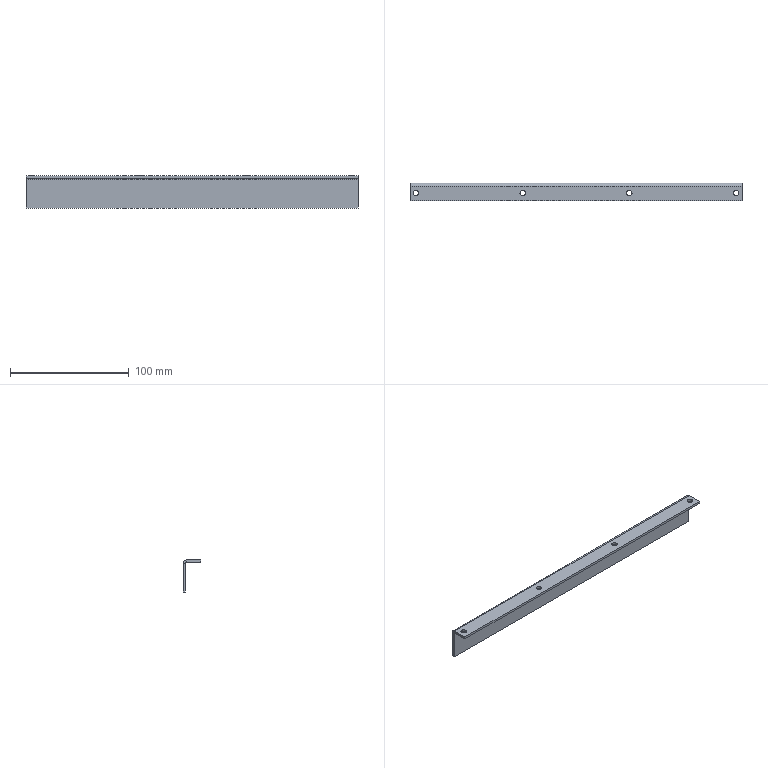Component | SolidWorks | P-SLJ-001-002-1 | 1 solid | 22 faces | box 280 x 15 x 27 mm | volume 21855 mm3 | plane 12 | cylinder 10 | commonest cylinder face diameters 4.5 x8 5.473 x1 1.473 x1 | material SUS 304
STEP:
#1=COLOUR_RGB('',0.7922,0.8196,0.9333);
#2=FILL_AREA_STYLE_COLOUR('',#1);
#3=FILL_AREA_STYLE('',(#2));
#4=SURFACE_STYLE_FILL_AREA(#3);
#5=SURFACE_SIDE_STYLE('',(#4));
#6=SURFACE_STYLE_USAGE(.BOTH.,#5);
#7=PRESENTATION_STYLE_ASSIGNMENT((#6));
#8=CARTESIAN_POINT('',(8.415,-2.579,48.253));
#9=VERTEX_POINT('',#8);
#10=CARTESIAN_POINT('',(8.238,-2.579,48.253));
#11=VERTEX_POINT('',#10);
#12=CARTESIAN_POINT('',(8.327,-2.579,48.253));
#13=DIRECTION('',(0.,0.,-1.));
#14=DIRECTION('',(-1.,0.,0.));
#15=AXIS2_PLACEMENT_3D('',#12,#13,#14);
#16=CIRCLE('',#15,0.08858);
#17=EDGE_CURVE('',#9,#11,#16,.T.);
#18=ORIENTED_EDGE('',*,*,#17,.F.);
#19=CARTESIAN_POINT('',(8.415,-2.579,48.175));
#20=VERTEX_POINT('',#19);
#21=CARTESIAN_POINT('',(8.415,-2.579,48.175));
#22=DIRECTION('',(0.,0.,-1.));
#23=VECTOR('',#22,39.37);
#24=LINE('',#21,#23);
#25=EDGE_CURVE('',#9,#20,#24,.T.);
#26=ORIENTED_EDGE('',*,*,#25,.T.);
#27=CARTESIAN_POINT('',(8.238,-2.579,48.175));
#28=VERTEX_POINT('',#27);
#29=CARTESIAN_POINT('',(8.327,-2.579,48.175));
#30=DIRECTION('',(0.,0.,-1.));
#31=DIRECTION('',(-1.,0.,0.));
#32=AXIS2_PLACEMENT_3D('',#29,#30,#31);
#33=CIRCLE('',#32,0.08858);
#34=EDGE_CURVE('',#20,#28,#33,.T.);
#35=ORIENTED_EDGE('',*,*,#34,.T.);
#36=CARTESIAN_POINT('',(8.238,-2.579,48.175));
#37=DIRECTION('',(0.,0.,-1.));
#38=VECTOR('',#37,39.37);
#39=LINE('',#36,#38);
#40=EDGE_CURVE('',#11,#28,#39,.T.);
#41=ORIENTED_EDGE('',*,*,#40,.F.);
#42=EDGE_LOOP('',(#18,#26,#35,#41));
#43=FACE_OUTER_BOUND('',#42,.T.);
#44=CARTESIAN_POINT('',(8.327,-2.579,48.175));
#45=DIRECTION('',(0.,0.,-1.));
#46=DIRECTION('',(-1.,0.,0.));
#47=AXIS2_PLACEMENT_3D('',#44,#45,#46);
#48=CYLINDRICAL_SURFACE('',#47,0.08858);
#49=ADVANCED_FACE('',(#43),#48,.F.);
#50=CARTESIAN_POINT('',(4.872,-2.579,48.253));
#51=VERTEX_POINT('',#50);
#52=CARTESIAN_POINT('',(4.695,-2.579,48.253));
#53=VERTEX_POINT('',#52);
#54=CARTESIAN_POINT('',(4.783,-2.579,48.253));
#55=DIRECTION('',(0.,0.,-1.));
#56=DIRECTION('',(-1.,0.,0.));
#57=AXIS2_PLACEMENT_3D('',#54,#55,#56);
#58=CIRCLE('',#57,0.08858);
#59=EDGE_CURVE('',#51,#53,#58,.T.);
#60=ORIENTED_EDGE('',*,*,#59,.F.);
#61=CARTESIAN_POINT('',(4.872,-2.579,48.175));
#62=VERTEX_POINT('',#61);
#63=CARTESIAN_POINT('',(4.872,-2.579,48.175));
#64=DIRECTION('',(0.,0.,-1.));
#65=VECTOR('',#64,39.37);
#66=LINE('',#63,#65);
#67=EDGE_CURVE('',#51,#62,#66,.T.);
#68=ORIENTED_EDGE('',*,*,#67,.T.);
#69=CARTESIAN_POINT('',(4.695,-2.579,48.175));
#70=VERTEX_POINT('',#69);
#71=CARTESIAN_POINT('',(4.783,-2.579,48.175));
#72=DIRECTION('',(0.,0.,-1.));
#73=DIRECTION('',(-1.,0.,0.));
#74=AXIS2_PLACEMENT_3D('',#71,#72,#73);
#75=CIRCLE('',#74,0.08858);
#76=EDGE_CURVE('',#62,#70,#75,.T.);
#77=ORIENTED_EDGE('',*,*,#76,.T.);
#78=CARTESIAN_POINT('',(4.695,-2.579,48.175));
#79=DIRECTION('',(0.,0.,-1.));
#80=VECTOR('',#79,39.37);
#81=LINE('',#78,#80);
#82=EDGE_CURVE('',#53,#70,#81,.T.);
#83=ORIENTED_EDGE('',*,*,#82,.F.);
#84=EDGE_LOOP('',(#60,#68,#77,#83));
#85=FACE_OUTER_BOUND('',#84,.T.);
#86=CARTESIAN_POINT('',(4.783,-2.579,48.175));
#87=DIRECTION('',(0.,0.,-1.));
#88=DIRECTION('',(-1.,0.,0.));
#89=AXIS2_PLACEMENT_3D('',#86,#87,#88);
#90=CYLINDRICAL_SURFACE('',#89,0.08858);
#91=ADVANCED_FACE('',(#85),#90,.F.);
#92=CARTESIAN_POINT('',(1.329,-2.579,48.253));
#93=VERTEX_POINT('',#92);
#94=CARTESIAN_POINT('',(1.152,-2.579,48.253));
#95=VERTEX_POINT('',#94);
#96=CARTESIAN_POINT('',(1.24,-2.579,48.253));
#97=DIRECTION('',(0.,0.,-1.));
#98=DIRECTION('',(-1.,0.,0.));
#99=AXIS2_PLACEMENT_3D('',#96,#97,#98);
#100=CIRCLE('',#99,0.08858);
#101=EDGE_CURVE('',#93,#95,#100,.T.);
#102=ORIENTED_EDGE('',*,*,#101,.F.);
#103=CARTESIAN_POINT('',(1.329,-2.579,48.175));
#104=VERTEX_POINT('',#103);
#105=CARTESIAN_POINT('',(1.329,-2.579,48.175));
#106=DIRECTION('',(0.,0.,-1.));
#107=VECTOR('',#106,39.37);
#108=LINE('',#105,#107);
#109=EDGE_CURVE('',#93,#104,#108,.T.);
#110=ORIENTED_EDGE('',*,*,#109,.T.);
#111=CARTESIAN_POINT('',(1.152,-2.579,48.175));
#112=VERTEX_POINT('',#111);
#113=CARTESIAN_POINT('',(1.24,-2.579,48.175));
#114=DIRECTION('',(0.,0.,-1.));
#115=DIRECTION('',(-1.,0.,0.));
#116=AXIS2_PLACEMENT_3D('',#113,#114,#115);
#117=CIRCLE('',#116,0.08858);
#118=EDGE_CURVE('',#104,#112,#117,.T.);
#119=ORIENTED_EDGE('',*,*,#118,.T.);
#120=CARTESIAN_POINT('',(1.152,-2.579,48.175));
#121=DIRECTION('',(0.,0.,-1.));
#122=VECTOR('',#121,39.37);
#123=LINE('',#120,#122);
#124=EDGE_CURVE('',#95,#112,#123,.T.);
#125=ORIENTED_EDGE('',*,*,#124,.F.);
#126=EDGE_LOOP('',(#102,#110,#119,#125));
#127=FACE_OUTER_BOUND('',#126,.T.);
#128=CARTESIAN_POINT('',(1.24,-2.579,48.175));
#129=DIRECTION('',(0.,0.,-1.));
#130=DIRECTION('',(-1.,0.,0.));
#131=AXIS2_PLACEMENT_3D('',#128,#129,#130);
#132=CYLINDRICAL_SURFACE('',#131,0.08858);
#133=ADVANCED_FACE('',(#127),#132,.F.);
#134=CARTESIAN_POINT('',(-2.215,-2.579,48.253));
#135=VERTEX_POINT('',#134);
#136=CARTESIAN_POINT('',(-2.392,-2.579,48.253));
#137=VERTEX_POINT('',#136);
#138=CARTESIAN_POINT('',(-2.303,-2.579,48.253));
#139=DIRECTION('',(0.,0.,-1.));
#140=DIRECTION('',(-1.,0.,0.));
#141=AXIS2_PLACEMENT_3D('',#138,#139,#140);
#142=CIRCLE('',#141,0.08858);
#143=EDGE_CURVE('',#135,#137,#142,.T.);
#144=ORIENTED_EDGE('',*,*,#143,.F.);
#145=CARTESIAN_POINT('',(-2.215,-2.579,48.175));
#146=VERTEX_POINT('',#145);
#147=CARTESIAN_POINT('',(-2.215,-2.579,48.175));
#148=DIRECTION('',(0.,0.,-1.));
#149=VECTOR('',#148,39.37);
#150=LINE('',#147,#149);
#151=EDGE_CURVE('',#135,#146,#150,.T.);
#152=ORIENTED_EDGE('',*,*,#151,.T.);
#153=CARTESIAN_POINT('',(-2.392,-2.579,48.175));
#154=VERTEX_POINT('',#153);
#155=CARTESIAN_POINT('',(-2.303,-2.579,48.175));
#156=DIRECTION('',(0.,0.,-1.));
#157=DIRECTION('',(-1.,0.,0.));
#158=AXIS2_PLACEMENT_3D('',#155,#156,#157);
#159=CIRCLE('',#158,0.08858);
#160=EDGE_CURVE('',#146,#154,#159,.T.);
#161=ORIENTED_EDGE('',*,*,#160,.T.);
#162=CARTESIAN_POINT('',(-2.392,-2.579,48.175));
#163=DIRECTION('',(0.,0.,-1.));
#164=VECTOR('',#163,39.37);
#165=LINE('',#162,#164);
#166=EDGE_CURVE('',#137,#154,#165,.T.);
#167=ORIENTED_EDGE('',*,*,#166,.F.);
#168=EDGE_LOOP('',(#144,#152,#161,#167));
#169=FACE_OUTER_BOUND('',#168,.T.);
#170=CARTESIAN_POINT('',(-2.303,-2.579,48.175));
#171=DIRECTION('',(0.,0.,-1.));
#172=DIRECTION('',(-1.,0.,0.));
#173=AXIS2_PLACEMENT_3D('',#170,#171,#172);
#174=CYLINDRICAL_SURFACE('',#173,0.08858);
#175=ADVANCED_FACE('',(#169),#174,.F.);
#176=CARTESIAN_POINT('',(8.524,-2.352,48.175));
#177=VERTEX_POINT('',#176);
#178=CARTESIAN_POINT('',(8.524,-2.835,48.175));
#179=VERTEX_POINT('',#178);
#180=CARTESIAN_POINT('',(8.524,-2.835,48.175));
#181=DIRECTION('',(-0.,-1.,0.));
#182=VECTOR('',#181,39.37);
#183=LINE('',#180,#182);
#184=EDGE_CURVE('',#177,#179,#183,.T.);
#185=ORIENTED_EDGE('',*,*,#184,.F.);
#186=CARTESIAN_POINT('',(8.524,-2.352,48.253));
#187=VERTEX_POINT('',#186);
#188=CARTESIAN_POINT('',(8.524,-2.352,48.175));
#189=DIRECTION('',(0.,0.,1.));
#190=VECTOR('',#189,39.37);
#191=LINE('',#188,#190);
#192=EDGE_CURVE('',#177,#187,#191,.T.);
#193=ORIENTED_EDGE('',*,*,#192,.T.);
#194=CARTESIAN_POINT('',(8.524,-2.835,48.253));
#195=VERTEX_POINT('',#194);
#196=CARTESIAN_POINT('',(8.524,-2.835,48.253));
#197=DIRECTION('',(-0.,-1.,0.));
#198=VECTOR('',#197,39.37);
#199=LINE('',#196,#198);
#200=EDGE_CURVE('',#187,#195,#199,.T.);
#201=ORIENTED_EDGE('',*,*,#200,.T.);
#202=CARTESIAN_POINT('',(8.524,-2.835,48.253));
#203=DIRECTION('',(0.,0.,-1.));
#204=VECTOR('',#203,39.37);
#205=LINE('',#202,#204);
#206=EDGE_CURVE('',#195,#179,#205,.T.);
#207=ORIENTED_EDGE('',*,*,#206,.T.);
#208=EDGE_LOOP('',(#185,#193,#201,#207));
#209=FACE_OUTER_BOUND('',#208,.T.);
#210=CARTESIAN_POINT('',(8.524,-2.835,48.253));
#211=DIRECTION('',(1.,-0.,0.));
#212=DIRECTION('',(0.,0.,-1.));
#213=AXIS2_PLACEMENT_3D('',#210,#211,#212);
#214=PLANE('',#213);
#215=ADVANCED_FACE('',(#209),#214,.T.);
#216=CARTESIAN_POINT('',(8.327,-2.579,48.253));
#217=DIRECTION('',(0.,0.,-1.));
#218=DIRECTION('',(-1.,0.,0.));
#219=AXIS2_PLACEMENT_3D('',#216,#217,#218);
#220=CIRCLE('',#219,0.08858);
#221=EDGE_CURVE('',#11,#9,#220,.T.);
#222=ORIENTED_EDGE('',*,*,#221,.T.);
#223=ORIENTED_EDGE('',*,*,#17,.T.);
#224=EDGE_LOOP('',(#222,#223));
#225=FACE_BOUND('',#224,.T.);
#226=CARTESIAN_POINT('',(4.783,-2.579,48.253));
#227=DIRECTION('',(0.,0.,-1.));
#228=DIRECTION('',(-1.,0.,0.));
#229=AXIS2_PLACEMENT_3D('',#226,#227,#228);
#230=CIRCLE('',#229,0.08858);
#231=EDGE_CURVE('',#53,#51,#230,.T.);
#232=ORIENTED_EDGE('',*,*,#231,.T.);
#233=ORIENTED_EDGE('',*,*,#59,.T.);
#234=EDGE_LOOP('',(#232,#233));
#235=FACE_BOUND('',#234,.T.);
#236=CARTESIAN_POINT('',(1.24,-2.579,48.253));
#237=DIRECTION('',(0.,0.,-1.));
#238=DIRECTION('',(-1.,0.,0.));
#239=AXIS2_PLACEMENT_3D('',#236,#237,#238);
#240=CIRCLE('',#239,0.08858);
#241=EDGE_CURVE('',#95,#93,#240,.T.);
#242=ORIENTED_EDGE('',*,*,#241,.T.);
#243=ORIENTED_EDGE('',*,*,#101,.T.);
#244=EDGE_LOOP('',(#242,#243));
#245=FACE_BOUND('',#244,.T.);
#246=CARTESIAN_POINT('',(-2.303,-2.579,48.253));
#247=DIRECTION('',(0.,0.,-1.));
#248=DIRECTION('',(-1.,0.,0.));
#249=AXIS2_PLACEMENT_3D('',#246,#247,#248);
#250=CIRCLE('',#249,0.08858);
#251=EDGE_CURVE('',#137,#135,#250,.T.);
#252=ORIENTED_EDGE('',*,*,#251,.T.);
#253=ORIENTED_EDGE('',*,*,#143,.T.);
#254=EDGE_LOOP('',(#252,#253));
#255=FACE_BOUND('',#254,.T.);
#256=ORIENTED_EDGE('',*,*,#200,.F.);
#257=CARTESIAN_POINT('',(-2.5,-2.352,48.253));
#258=VERTEX_POINT('',#257);
#259=CARTESIAN_POINT('',(8.524,-2.352,48.253));
#260=DIRECTION('',(-1.,0.,0.));
#261=VECTOR('',#260,39.37);
#262=LINE('',#259,#261);
#263=EDGE_CURVE('',#187,#258,#262,.T.);
#264=ORIENTED_EDGE('',*,*,#263,.T.);
#265=CARTESIAN_POINT('',(-2.5,-2.835,48.253));
#266=VERTEX_POINT('',#265);
#267=CARTESIAN_POINT('',(-2.5,-2.835,48.253));
#268=DIRECTION('',(0.,1.,0.));
#269=VECTOR('',#268,39.37);
#270=LINE('',#267,#269);
#271=EDGE_CURVE('',#266,#258,#270,.T.);
#272=ORIENTED_EDGE('',*,*,#271,.F.);
#273=CARTESIAN_POINT('',(8.524,-2.835,48.253));
#274=DIRECTION('',(-1.,0.,0.));
#275=VECTOR('',#274,39.37);
#276=LINE('',#273,#275);
#277=EDGE_CURVE('',#195,#266,#276,.T.);
#278=ORIENTED_EDGE('',*,*,#277,.F.);
#279=EDGE_LOOP('',(#256,#264,#272,#278));
#280=FACE_OUTER_BOUND('',#279,.T.);
#281=CARTESIAN_POINT('',(3.012,-2.579,48.253));
#282=DIRECTION('',(0.,0.,1.));
#283=DIRECTION('',(1.,-0.,0.));
#284=AXIS2_PLACEMENT_3D('',#281,#282,#283);
#285=PLANE('',#284);
#286=ADVANCED_FACE('',(#225,#235,#245,#255,#280),#285,.T.);
#287=CARTESIAN_POINT('',(8.327,-2.579,48.175));
#288=DIRECTION('',(0.,0.,-1.));
#289=DIRECTION('',(-1.,0.,0.));
#290=AXIS2_PLACEMENT_3D('',#287,#288,#289);
#291=CIRCLE('',#290,0.08858);
#292=EDGE_CURVE('',#28,#20,#291,.T.);
#293=ORIENTED_EDGE('',*,*,#292,.F.);
#294=ORIENTED_EDGE('',*,*,#34,.F.);
#295=EDGE_LOOP('',(#293,#294));
#296=FACE_BOUND('',#295,.T.);
#297=CARTESIAN_POINT('',(4.783,-2.579,48.175));
#298=DIRECTION('',(0.,0.,-1.));
#299=DIRECTION('',(-1.,0.,0.));
#300=AXIS2_PLACEMENT_3D('',#297,#298,#299);
#301=CIRCLE('',#300,0.08858);
#302=EDGE_CURVE('',#70,#62,#301,.T.);
#303=ORIENTED_EDGE('',*,*,#302,.F.);
#304=ORIENTED_EDGE('',*,*,#76,.F.);
#305=EDGE_LOOP('',(#303,#304));
#306=FACE_BOUND('',#305,.T.);
#307=CARTESIAN_POINT('',(1.24,-2.579,48.175));
#308=DIRECTION('',(0.,0.,-1.));
#309=DIRECTION('',(-1.,0.,0.));
#310=AXIS2_PLACEMENT_3D('',#307,#308,#309);
#311=CIRCLE('',#310,0.08858);
#312=EDGE_CURVE('',#112,#104,#311,.T.);
#313=ORIENTED_EDGE('',*,*,#312,.F.);
#314=ORIENTED_EDGE('',*,*,#118,.F.);
#315=EDGE_LOOP('',(#313,#314));
#316=FACE_BOUND('',#315,.T.);
#317=CARTESIAN_POINT('',(-2.303,-2.579,48.175));
#318=DIRECTION('',(0.,0.,-1.));
#319=DIRECTION('',(-1.,0.,0.));
#320=AXIS2_PLACEMENT_3D('',#317,#318,#319);
#321=CIRCLE('',#320,0.08858);
#322=EDGE_CURVE('',#154,#146,#321,.T.);
#323=ORIENTED_EDGE('',*,*,#322,.F.);
#324=ORIENTED_EDGE('',*,*,#160,.F.);
#325=EDGE_LOOP('',(#323,#324));
#326=FACE_BOUND('',#325,.T.);
#327=CARTESIAN_POINT('',(-2.5,-2.352,48.175));
#328=VERTEX_POINT('',#327);
#329=CARTESIAN_POINT('',(8.524,-2.352,48.175));
#330=DIRECTION('',(-1.,0.,0.));
#331=VECTOR('',#330,39.37);
#332=LINE('',#329,#331);
#333=EDGE_CURVE('',#177,#328,#332,.T.);
#334=ORIENTED_EDGE('',*,*,#333,.F.);
#335=ORIENTED_EDGE('',*,*,#184,.T.);
#336=CARTESIAN_POINT('',(-2.5,-2.835,48.175));
#337=VERTEX_POINT('',#336);
#338=CARTESIAN_POINT('',(8.524,-2.835,48.175));
#339=DIRECTION('',(-1.,0.,0.));
#340=VECTOR('',#339,39.37);
#341=LINE('',#338,#340);
#342=EDGE_CURVE('',#179,#337,#341,.T.);
#343=ORIENTED_EDGE('',*,*,#342,.T.);
#344=CARTESIAN_POINT('',(-2.5,-2.835,48.175));
#345=DIRECTION('',(0.,1.,0.));
#346=VECTOR('',#345,39.37);
#347=LINE('',#344,#346);
#348=EDGE_CURVE('',#337,#328,#347,.T.);
#349=ORIENTED_EDGE('',*,*,#348,.T.);
#350=EDGE_LOOP('',(#334,#335,#343,#349));
#351=FACE_OUTER_BOUND('',#350,.T.);
#352=CARTESIAN_POINT('',(3.012,-2.579,48.175));
#353=DIRECTION('',(0.,0.,1.));
#354=DIRECTION('',(1.,-0.,0.));
#355=AXIS2_PLACEMENT_3D('',#352,#353,#354);
#356=PLANE('',#355);
#357=ADVANCED_FACE('',(#296,#306,#316,#326,#351),#356,.F.);
#358=CARTESIAN_POINT('',(-2.5,-2.352,48.175));
#359=DIRECTION('',(0.,0.,1.));
#360=VECTOR('',#359,39.37);
#361=LINE('',#358,#360);
#362=EDGE_CURVE('',#328,#258,#361,.T.);
#363=ORIENTED_EDGE('',*,*,#362,.F.);
#364=ORIENTED_EDGE('',*,*,#348,.F.);
#365=CARTESIAN_POINT('',(-2.5,-2.835,48.253));
#366=DIRECTION('',(0.,0.,-1.));
#367=VECTOR('',#366,39.37);
#368=LINE('',#365,#367);
#369=EDGE_CURVE('',#266,#337,#368,.T.);
#370=ORIENTED_EDGE('',*,*,#369,.F.);
#371=ORIENTED_EDGE('',*,*,#271,.T.);
#372=EDGE_LOOP('',(#363,#364,#370,#371));
#373=FACE_OUTER_BOUND('',#372,.T.);
#374=CARTESIAN_POINT('',(-2.5,-2.835,48.253));
#375=DIRECTION('',(-1.,0.,0.));
#376=DIRECTION('',(0.,0.,1.));
#377=AXIS2_PLACEMENT_3D('',#374,#375,#376);
#378=PLANE('',#377);
#379=ADVANCED_FACE('',(#373),#378,.T.);
#380=ORIENTED_EDGE('',*,*,#342,.F.);
#381=ORIENTED_EDGE('',*,*,#206,.F.);
#382=ORIENTED_EDGE('',*,*,#277,.T.);
#383=ORIENTED_EDGE('',*,*,#369,.T.);
#384=EDGE_LOOP('',(#380,#381,#382,#383));
#385=FACE_OUTER_BOUND('',#384,.T.);
#386=CARTESIAN_POINT('',(8.524,-2.835,48.253));
#387=DIRECTION('',(-0.,-1.,0.));
#388=DIRECTION('',(-1.,0.,0.));
#389=AXIS2_PLACEMENT_3D('',#386,#387,#388);
#390=PLANE('',#389);
#391=ADVANCED_FACE('',(#385),#390,.T.);
#392=CARTESIAN_POINT('',(-2.5,-2.323,48.146));
#393=VERTEX_POINT('',#392);
#394=CARTESIAN_POINT('',(-2.5,-2.244,48.146));
#395=VERTEX_POINT('',#394);
#396=CARTESIAN_POINT('',(-2.5,-2.323,48.146));
#397=DIRECTION('',(0.,1.,0.));
#398=VECTOR('',#397,39.37);
#399=LINE('',#396,#398);
#400=EDGE_CURVE('',#393,#395,#399,.T.);
#401=ORIENTED_EDGE('',*,*,#400,.F.);
#402=CARTESIAN_POINT('',(-2.5,-2.352,48.146));
#403=DIRECTION('',(-1.,0.,0.));
#404=DIRECTION('',(0.,0.,-1.));
#405=AXIS2_PLACEMENT_3D('',#402,#403,#404);
#406=CIRCLE('',#405,0.029);
#407=EDGE_CURVE('',#328,#393,#406,.T.);
#408=ORIENTED_EDGE('',*,*,#407,.F.);
#409=ORIENTED_EDGE('',*,*,#362,.T.);
#410=CARTESIAN_POINT('',(-2.5,-2.352,48.146));
#411=DIRECTION('',(-1.,0.,0.));
#412=DIRECTION('',(0.,0.,-1.));
#413=AXIS2_PLACEMENT_3D('',#410,#411,#412);
#414=CIRCLE('',#413,0.1077);
#415=EDGE_CURVE('',#258,#395,#414,.T.);
#416=ORIENTED_EDGE('',*,*,#415,.T.);
#417=EDGE_LOOP('',(#401,#408,#409,#416));
#418=FACE_OUTER_BOUND('',#417,.T.);
#419=CARTESIAN_POINT('',(-2.5,-2.352,48.146));
#420=DIRECTION('',(-1.,0.,0.));
#421=DIRECTION('',(0.,0.,1.));
#422=AXIS2_PLACEMENT_3D('',#419,#420,#421);
#423=PLANE('',#422);
#424=ADVANCED_FACE('',(#418),#423,.T.);
#425=CARTESIAN_POINT('',(8.524,-2.323,48.146));
#426=VERTEX_POINT('',#425);
#427=CARTESIAN_POINT('',(8.524,-2.352,48.146));
#428=DIRECTION('',(1.,-0.,0.));
#429=DIRECTION('',(0.,0.,-1.));
#430=AXIS2_PLACEMENT_3D('',#427,#428,#429);
#431=CIRCLE('',#430,0.029);
#432=EDGE_CURVE('',#426,#177,#431,.T.);
#433=ORIENTED_EDGE('',*,*,#432,.F.);
#434=CARTESIAN_POINT('',(8.524,-2.244,48.146));
#435=VERTEX_POINT('',#434);
#436=CARTESIAN_POINT('',(8.524,-2.323,48.146));
#437=DIRECTION('',(0.,1.,0.));
#438=VECTOR('',#437,39.37);
#439=LINE('',#436,#438);
#440=EDGE_CURVE('',#426,#435,#439,.T.);
#441=ORIENTED_EDGE('',*,*,#440,.T.);
#442=CARTESIAN_POINT('',(8.524,-2.352,48.146));
#443=DIRECTION('',(1.,-0.,0.));
#444=DIRECTION('',(0.,0.,-1.));
#445=AXIS2_PLACEMENT_3D('',#442,#443,#444);
#446=CIRCLE('',#445,0.1077);
#447=EDGE_CURVE('',#435,#187,#446,.T.);
#448=ORIENTED_EDGE('',*,*,#447,.T.);
#449=ORIENTED_EDGE('',*,*,#192,.F.);
#450=EDGE_LOOP('',(#433,#441,#448,#449));
#451=FACE_OUTER_BOUND('',#450,.T.);
#452=CARTESIAN_POINT('',(8.524,-2.352,48.146));
#453=DIRECTION('',(-1.,0.,0.));
#454=DIRECTION('',(0.,0.,1.));
#455=AXIS2_PLACEMENT_3D('',#452,#453,#454);
#456=PLANE('',#455);
#457=ADVANCED_FACE('',(#451),#456,.F.);
#458=ORIENTED_EDGE('',*,*,#263,.F.);
#459=ORIENTED_EDGE('',*,*,#447,.F.);
#460=CARTESIAN_POINT('',(3.012,-2.244,48.146));
#461=DIRECTION('',(-1.,0.,0.));
#462=VECTOR('',#461,39.37);
#463=LINE('',#460,#462);
#464=EDGE_CURVE('',#435,#395,#463,.T.);
#465=ORIENTED_EDGE('',*,*,#464,.T.);
#466=ORIENTED_EDGE('',*,*,#415,.F.);
#467=EDGE_LOOP('',(#458,#459,#465,#466));
#468=FACE_OUTER_BOUND('',#467,.T.);
#469=CARTESIAN_POINT('',(8.524,-2.352,48.146));
#470=DIRECTION('',(1.,-0.,0.));
#471=DIRECTION('',(0.,1.,0.));
#472=AXIS2_PLACEMENT_3D('',#469,#470,#471);
#473=CYLINDRICAL_SURFACE('',#472,0.1077);
#474=ADVANCED_FACE('',(#468),#473,.T.);
#475=ORIENTED_EDGE('',*,*,#333,.T.);
#476=ORIENTED_EDGE('',*,*,#407,.T.);
#477=CARTESIAN_POINT('',(-2.5,-2.323,48.146));
#478=DIRECTION('',(1.,-0.,-0.));
#479=VECTOR('',#478,39.37);
#480=LINE('',#477,#479);
#481=EDGE_CURVE('',#393,#426,#480,.T.);
#482=ORIENTED_EDGE('',*,*,#481,.T.);
#483=ORIENTED_EDGE('',*,*,#432,.T.);
#484=EDGE_LOOP('',(#475,#476,#482,#483));
#485=FACE_OUTER_BOUND('',#484,.T.);
#486=CARTESIAN_POINT('',(8.524,-2.352,48.146));
#487=DIRECTION('',(1.,-0.,0.));
#488=DIRECTION('',(0.,1.,0.));
#489=AXIS2_PLACEMENT_3D('',#486,#487,#488);
#490=CYLINDRICAL_SURFACE('',#489,0.029);
#491=ADVANCED_FACE('',(#485),#490,.F.);
#492=ORIENTED_EDGE('',*,*,#440,.F.);
#493=CARTESIAN_POINT('',(8.524,-2.323,47.19));
#494=VERTEX_POINT('',#493);
#495=CARTESIAN_POINT('',(8.524,-2.323,47.19));
#496=DIRECTION('',(0.,0.,-1.));
#497=VECTOR('',#496,39.37);
#498=LINE('',#495,#497);
#499=EDGE_CURVE('',#426,#494,#498,.T.);
#500=ORIENTED_EDGE('',*,*,#499,.T.);
#501=CARTESIAN_POINT('',(8.524,-2.244,47.19));
#502=VERTEX_POINT('',#501);
#503=CARTESIAN_POINT('',(8.524,-2.244,47.19));
#504=DIRECTION('',(-0.,-1.,-0.));
#505=VECTOR('',#504,39.37);
#506=LINE('',#503,#505);
#507=EDGE_CURVE('',#502,#494,#506,.T.);
#508=ORIENTED_EDGE('',*,*,#507,.F.);
#509=CARTESIAN_POINT('',(8.524,-2.244,47.19));
#510=DIRECTION('',(0.,0.,-1.));
#511=VECTOR('',#510,39.37);
#512=LINE('',#509,#511);
#513=EDGE_CURVE('',#435,#502,#512,.T.);
#514=ORIENTED_EDGE('',*,*,#513,.F.);
#515=EDGE_LOOP('',(#492,#500,#508,#514));
#516=FACE_OUTER_BOUND('',#515,.T.);
#517=CARTESIAN_POINT('',(8.524,-2.244,47.19));
#518=DIRECTION('',(-1.,0.,0.));
#519=DIRECTION('',(0.,0.,1.));
#520=AXIS2_PLACEMENT_3D('',#517,#518,#519);
#521=PLANE('',#520);
#522=ADVANCED_FACE('',(#516),#521,.F.);
#523=ORIENTED_EDGE('',*,*,#400,.T.);
#524=CARTESIAN_POINT('',(-2.5,-2.244,47.19));
#525=VERTEX_POINT('',#524);
#526=CARTESIAN_POINT('',(-2.5,-2.244,48.175));
#527=DIRECTION('',(-0.,-0.,1.));
#528=VECTOR('',#527,39.37);
#529=LINE('',#526,#528);
#530=EDGE_CURVE('',#525,#395,#529,.T.);
#531=ORIENTED_EDGE('',*,*,#530,.F.);
#532=CARTESIAN_POINT('',(-2.5,-2.323,47.19));
#533=VERTEX_POINT('',#532);
#534=CARTESIAN_POINT('',(-2.5,-2.244,47.19));
#535=DIRECTION('',(-0.,-1.,-0.));
#536=VECTOR('',#535,39.37);
#537=LINE('',#534,#536);
#538=EDGE_CURVE('',#525,#533,#537,.T.);
#539=ORIENTED_EDGE('',*,*,#538,.T.);
#540=CARTESIAN_POINT('',(-2.5,-2.323,48.175));
#541=DIRECTION('',(-0.,-0.,1.));
#542=VECTOR('',#541,39.37);
#543=LINE('',#540,#542);
#544=EDGE_CURVE('',#533,#393,#543,.T.);
#545=ORIENTED_EDGE('',*,*,#544,.T.);
#546=EDGE_LOOP('',(#523,#531,#539,#545));
#547=FACE_OUTER_BOUND('',#546,.T.);
#548=CARTESIAN_POINT('',(-2.5,-2.244,48.175));
#549=DIRECTION('',(1.,-0.,0.));
#550=DIRECTION('',(0.,0.,-1.));
#551=AXIS2_PLACEMENT_3D('',#548,#549,#550);
#552=PLANE('',#551);
#553=ADVANCED_FACE('',(#547),#552,.F.);
#554=ORIENTED_EDGE('',*,*,#464,.F.);
#555=ORIENTED_EDGE('',*,*,#513,.T.);
#556=CARTESIAN_POINT('',(-2.5,-2.244,47.19));
#557=DIRECTION('',(-1.,0.,0.));
#558=VECTOR('',#557,39.37);
#559=LINE('',#556,#558);
#560=EDGE_CURVE('',#502,#525,#559,.T.);
#561=ORIENTED_EDGE('',*,*,#560,.T.);
#562=ORIENTED_EDGE('',*,*,#530,.T.);
#563=EDGE_LOOP('',(#554,#555,#561,#562));
#564=FACE_OUTER_BOUND('',#563,.T.);
#565=CARTESIAN_POINT('',(3.012,-2.244,48.175));
#566=DIRECTION('',(-0.,-1.,-0.));
#567=DIRECTION('',(0.,0.,-1.));
#568=AXIS2_PLACEMENT_3D('',#565,#566,#567);
#569=PLANE('',#568);
#570=ADVANCED_FACE('',(#564),#569,.F.);
#571=ORIENTED_EDGE('',*,*,#499,.F.);
#572=ORIENTED_EDGE('',*,*,#481,.F.);
#573=ORIENTED_EDGE('',*,*,#544,.F.);
#574=CARTESIAN_POINT('',(-2.5,-2.323,47.19));
#575=DIRECTION('',(-1.,0.,0.));
#576=VECTOR('',#575,39.37);
#577=LINE('',#574,#576);
#578=EDGE_CURVE('',#494,#533,#577,.T.);
#579=ORIENTED_EDGE('',*,*,#578,.F.);
#580=EDGE_LOOP('',(#571,#572,#573,#579));
#581=FACE_OUTER_BOUND('',#580,.T.);
#582=CARTESIAN_POINT('',(3.012,-2.323,48.175));
#583=DIRECTION('',(-0.,-1.,-0.));
#584=DIRECTION('',(0.,0.,-1.));
#585=AXIS2_PLACEMENT_3D('',#582,#583,#584);
#586=PLANE('',#585);
#587=ADVANCED_FACE('',(#581),#586,.T.);
#588=ORIENTED_EDGE('',*,*,#578,.T.);
#589=ORIENTED_EDGE('',*,*,#538,.F.);
#590=ORIENTED_EDGE('',*,*,#560,.F.);
#591=ORIENTED_EDGE('',*,*,#507,.T.);
#592=EDGE_LOOP('',(#588,#589,#590,#591));
#593=FACE_OUTER_BOUND('',#592,.T.);
#594=CARTESIAN_POINT('',(-2.5,-2.244,47.19));
#595=DIRECTION('',(-0.,-0.,1.));
#596=DIRECTION('',(-0.,-1.,-0.));
#597=AXIS2_PLACEMENT_3D('',#594,#595,#596);
#598=PLANE('',#597);
#599=ADVANCED_FACE('',(#593),#598,.F.);
#600=ORIENTED_EDGE('',*,*,#151,.F.);
#601=ORIENTED_EDGE('',*,*,#251,.F.);
#602=ORIENTED_EDGE('',*,*,#166,.T.);
#603=ORIENTED_EDGE('',*,*,#322,.T.);
#604=EDGE_LOOP('',(#600,#601,#602,#603));
#605=FACE_OUTER_BOUND('',#604,.T.);
#606=CARTESIAN_POINT('',(-2.303,-2.579,48.175));
#607=DIRECTION('',(0.,0.,-1.));
#608=DIRECTION('',(-1.,0.,0.));
#609=AXIS2_PLACEMENT_3D('',#606,#607,#608);
#610=CYLINDRICAL_SURFACE('',#609,0.08858);
#611=ADVANCED_FACE('',(#605),#610,.F.);
#612=ORIENTED_EDGE('',*,*,#109,.F.);
#613=ORIENTED_EDGE('',*,*,#241,.F.);
#614=ORIENTED_EDGE('',*,*,#124,.T.);
#615=ORIENTED_EDGE('',*,*,#312,.T.);
#616=EDGE_LOOP('',(#612,#613,#614,#615));
#617=FACE_OUTER_BOUND('',#616,.T.);
#618=CARTESIAN_POINT('',(1.24,-2.579,48.175));
#619=DIRECTION('',(0.,0.,-1.));
#620=DIRECTION('',(-1.,0.,0.));
#621=AXIS2_PLACEMENT_3D('',#618,#619,#620);
#622=CYLINDRICAL_SURFACE('',#621,0.08858);
#623=ADVANCED_FACE('',(#617),#622,.F.);
#624=ORIENTED_EDGE('',*,*,#67,.F.);
#625=ORIENTED_EDGE('',*,*,#231,.F.);
#626=ORIENTED_EDGE('',*,*,#82,.T.);
#627=ORIENTED_EDGE('',*,*,#302,.T.);
#628=EDGE_LOOP('',(#624,#625,#626,#627));
#629=FACE_OUTER_BOUND('',#628,.T.);
#630=CARTESIAN_POINT('',(4.783,-2.579,48.175));
#631=DIRECTION('',(0.,0.,-1.));
#632=DIRECTION('',(-1.,0.,0.));
#633=AXIS2_PLACEMENT_3D('',#630,#631,#632);
#634=CYLINDRICAL_SURFACE('',#633,0.08858);
#635=ADVANCED_FACE('',(#629),#634,.F.);
#636=ORIENTED_EDGE('',*,*,#25,.F.);
#637=ORIENTED_EDGE('',*,*,#221,.F.);
#638=ORIENTED_EDGE('',*,*,#40,.T.);
#639=ORIENTED_EDGE('',*,*,#292,.T.);
#640=EDGE_LOOP('',(#636,#637,#638,#639));
#641=FACE_OUTER_BOUND('',#640,.T.);
#642=CARTESIAN_POINT('',(8.327,-2.579,48.175));
#643=DIRECTION('',(0.,0.,-1.));
#644=DIRECTION('',(-1.,0.,0.));
#645=AXIS2_PLACEMENT_3D('',#642,#643,#644);
#646=CYLINDRICAL_SURFACE('',#645,0.08858);
#647=ADVANCED_FACE('',(#641),#646,.F.);
#648=CLOSED_SHELL('',(#49,#91,#133,#175,#215,#286,#357,#379,#391,#424,#457,#474,#491,#522,#553,#570,#587,#599,#611,#623,#635,#647));
#649=MANIFOLD_SOLID_BREP('',#648);
#650=STYLED_ITEM('',(#7),#649);
#651=(LENGTH_UNIT()NAMED_UNIT(*)SI_UNIT($,.METRE.));
#652=LENGTH_MEASURE_WITH_UNIT(LENGTH_MEASURE(0.0254),#651);
#653=DIMENSIONAL_EXPONENTS(1.,0.,0.,0.,0.,0.,0.);
#654=(CONVERSION_BASED_UNIT('',#652)LENGTH_UNIT()NAMED_UNIT(#653));
#655=UNCERTAINTY_MEASURE_WITH_UNIT(LENGTH_MEASURE(0.00001),#654,'','');
#656=(NAMED_UNIT(*)PLANE_ANGLE_UNIT()SI_UNIT($,.RADIAN.));
#657=(NAMED_UNIT(*)SI_UNIT($,.STERADIAN.)SOLID_ANGLE_UNIT());
#658=(GEOMETRIC_REPRESENTATION_CONTEXT(3)GLOBAL_UNCERTAINTY_ASSIGNED_CONTEXT((#655))GLOBAL_UNIT_ASSIGNED_CONTEXT((#654,#656,#657))REPRESENTATION_CONTEXT('',''));
#659=MECHANICAL_DESIGN_GEOMETRIC_PRESENTATION_REPRESENTATION('',(#650),#658);
#660=CARTESIAN_POINT('',(0.,0.,0.));
#661=DIRECTION('',(0.,0.,1.));
#662=DIRECTION('',(1.,0.,0.));
#663=AXIS2_PLACEMENT_3D('',#660,#661,#662);
#664=(LENGTH_UNIT()NAMED_UNIT(*)SI_UNIT($,.METRE.));
#665=LENGTH_MEASURE_WITH_UNIT(LENGTH_MEASURE(0.0254),#664);
#666=DIMENSIONAL_EXPONENTS(1.,0.,0.,0.,0.,0.,0.);
#667=(CONVERSION_BASED_UNIT('',#665)LENGTH_UNIT()NAMED_UNIT(#666));
#668=UNCERTAINTY_MEASURE_WITH_UNIT(LENGTH_MEASURE(0.00001),#667,'','');
#669=(NAMED_UNIT(*)PLANE_ANGLE_UNIT()SI_UNIT($,.RADIAN.));
#670=(NAMED_UNIT(*)SI_UNIT($,.STERADIAN.)SOLID_ANGLE_UNIT());
#671=(GEOMETRIC_REPRESENTATION_CONTEXT(3)GLOBAL_UNCERTAINTY_ASSIGNED_CONTEXT((#668))GLOBAL_UNIT_ASSIGNED_CONTEXT((#667,#669,#670))REPRESENTATION_CONTEXT('',''));
#672=ADVANCED_BREP_SHAPE_REPRESENTATION('',(#649,#663),#671);
#673=PRESENTATION_LAYER_ASSIGNMENT('','',(#650));